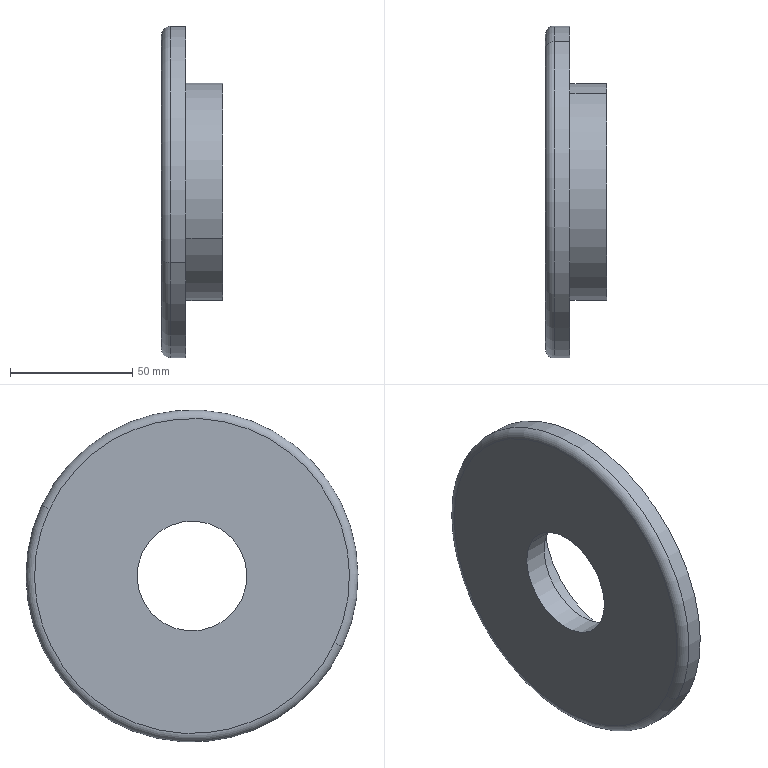Component | SolidWorks | LowerEndCap-1 | 1 solid | 14 faces | box 25 x 136 x 136 mm | volume 155302 mm3 | cylinder 8 | plane 4 | torus 2 | commonest cylinder face diameters 45 x2 75 x2 89 x2 136 x2
build123d program:
from build123d import *


with BuildPart() as part:
    # Sketch1 → Revolve1 (revolve)
    with BuildSketch(Plane(origin=(0, 0, 0), x_dir=(0, 0, -1), z_dir=(1, 0, 0)), mode=Mode.PRIVATE) as revolve1_sk:
        with BuildLine():
            Line((22.5, -10), (64.5, -10))
            ThreePointArc((64.5, -10), (66.975, -8.975), (68, -6.5))
            Line((68, -6.5), (68, 0))
            Line((68, 0), (44.5, 0))
            Line((44.5, 0), (44.5, 15))
            Line((44.5, 15), (37.5, 15))
            Line((37.5, 15), (37.5, 0))
            Line((37.5, 0), (22.5, 0))
            Line((22.5, 0), (22.5, -10))
        make_face()
    revolve(revolve1_sk.sketch.rotate(Axis((0, 0, 0), (0, -1, 0)), 180), axis=Axis((0, 0, 0), (0, -1, 0)))


solid = part.part

# Placed as in the assembly
solid = solid.moved(Location((587.733, 15.31, -110), (0, 0, -90)))
STEP:
#1=COLOUR_RGB('',0.7922,0.8196,0.9333);
#2=FILL_AREA_STYLE_COLOUR('',#1);
#3=FILL_AREA_STYLE('',(#2));
#4=SURFACE_STYLE_FILL_AREA(#3);
#5=SURFACE_SIDE_STYLE('',(#4));
#6=SURFACE_STYLE_USAGE(.BOTH.,#5);
#7=PRESENTATION_STYLE_ASSIGNMENT((#6));
#8=CARTESIAN_POINT('',(22.745,1.405,-3.955));
#9=VERTEX_POINT('',#8);
#10=CARTESIAN_POINT('',(22.745,-0.1993,-4.707));
#11=VERTEX_POINT('',#10);
#12=CARTESIAN_POINT('',(22.745,0.6028,-4.331));
#13=DIRECTION('',(1.,0.,0.));
#14=DIRECTION('',(0.,-0.9054,-0.4246));
#15=AXIS2_PLACEMENT_3D('',#12,#13,#14);
#16=CIRCLE('',#15,0.8858);
#17=EDGE_CURVE('',#9,#11,#16,.T.);
#18=ORIENTED_EDGE('',*,*,#17,.F.);
#19=CARTESIAN_POINT('',(23.139,1.405,-3.955));
#20=VERTEX_POINT('',#19);
#21=CARTESIAN_POINT('',(23.139,1.405,-3.955));
#22=DIRECTION('',(1.,0.,0.));
#23=VECTOR('',#22,39.37);
#24=LINE('',#21,#23);
#25=EDGE_CURVE('',#9,#20,#24,.T.);
#26=ORIENTED_EDGE('',*,*,#25,.T.);
#27=CARTESIAN_POINT('',(23.139,-0.1993,-4.707));
#28=VERTEX_POINT('',#27);
#29=CARTESIAN_POINT('',(23.139,0.6028,-4.331));
#30=DIRECTION('',(1.,0.,0.));
#31=DIRECTION('',(0.,-0.9054,-0.4246));
#32=AXIS2_PLACEMENT_3D('',#29,#30,#31);
#33=CIRCLE('',#32,0.8858);
#34=EDGE_CURVE('',#20,#28,#33,.T.);
#35=ORIENTED_EDGE('',*,*,#34,.T.);
#36=CARTESIAN_POINT('',(23.139,-0.1993,-4.707));
#37=DIRECTION('',(1.,0.,0.));
#38=VECTOR('',#37,39.37);
#39=LINE('',#36,#38);
#40=EDGE_CURVE('',#11,#28,#39,.T.);
#41=ORIENTED_EDGE('',*,*,#40,.F.);
#42=EDGE_LOOP('',(#18,#26,#35,#41));
#43=FACE_OUTER_BOUND('',#42,.T.);
#44=CARTESIAN_POINT('',(23.139,0.6028,-4.331));
#45=DIRECTION('',(1.,0.,0.));
#46=DIRECTION('',(0.,-0.9054,-0.4246));
#47=AXIS2_PLACEMENT_3D('',#44,#45,#46);
#48=CYLINDRICAL_SURFACE('',#47,0.8858);
#49=ADVANCED_FACE('',(#43),#48,.F.);
#50=CARTESIAN_POINT('',(23.139,1.939,-3.704));
#51=VERTEX_POINT('',#50);
#52=CARTESIAN_POINT('',(23.139,-0.7339,-4.958));
#53=VERTEX_POINT('',#52);
#54=CARTESIAN_POINT('',(23.139,0.6028,-4.331));
#55=DIRECTION('',(1.,0.,0.));
#56=DIRECTION('',(0.,-0.9054,-0.4246));
#57=AXIS2_PLACEMENT_3D('',#54,#55,#56);
#58=CIRCLE('',#57,1.476);
#59=EDGE_CURVE('',#51,#53,#58,.T.);
#60=ORIENTED_EDGE('',*,*,#59,.F.);
#61=CARTESIAN_POINT('',(23.73,1.939,-3.704));
#62=VERTEX_POINT('',#61);
#63=CARTESIAN_POINT('',(23.139,1.939,-3.704));
#64=DIRECTION('',(1.,0.,0.));
#65=VECTOR('',#64,39.37);
#66=LINE('',#63,#65);
#67=EDGE_CURVE('',#51,#62,#66,.T.);
#68=ORIENTED_EDGE('',*,*,#67,.T.);
#69=CARTESIAN_POINT('',(23.73,-0.7339,-4.958));
#70=VERTEX_POINT('',#69);
#71=CARTESIAN_POINT('',(23.73,0.6028,-4.331));
#72=DIRECTION('',(1.,0.,0.));
#73=DIRECTION('',(0.,-0.9054,-0.4246));
#74=AXIS2_PLACEMENT_3D('',#71,#72,#73);
#75=CIRCLE('',#74,1.476);
#76=EDGE_CURVE('',#62,#70,#75,.T.);
#77=ORIENTED_EDGE('',*,*,#76,.T.);
#78=CARTESIAN_POINT('',(23.139,-0.7339,-4.958));
#79=DIRECTION('',(1.,0.,0.));
#80=VECTOR('',#79,39.37);
#81=LINE('',#78,#80);
#82=EDGE_CURVE('',#53,#70,#81,.T.);
#83=ORIENTED_EDGE('',*,*,#82,.F.);
#84=EDGE_LOOP('',(#60,#68,#77,#83));
#85=FACE_OUTER_BOUND('',#84,.T.);
#86=CARTESIAN_POINT('',(23.139,0.6028,-4.331));
#87=DIRECTION('',(1.,0.,0.));
#88=DIRECTION('',(0.,-0.9054,-0.4246));
#89=AXIS2_PLACEMENT_3D('',#86,#87,#88);
#90=CYLINDRICAL_SURFACE('',#89,1.476);
#91=ADVANCED_FACE('',(#85),#90,.F.);
#92=CARTESIAN_POINT('',(23.139,-0.9835,-5.075));
#93=VERTEX_POINT('',#92);
#94=CARTESIAN_POINT('',(23.139,2.189,-3.587));
#95=VERTEX_POINT('',#94);
#96=CARTESIAN_POINT('',(23.139,0.6028,-4.331));
#97=DIRECTION('',(1.,0.,0.));
#98=DIRECTION('',(0.,-0.9054,-0.4246));
#99=AXIS2_PLACEMENT_3D('',#96,#97,#98);
#100=CIRCLE('',#99,1.752);
#101=EDGE_CURVE('',#93,#95,#100,.T.);
#102=ORIENTED_EDGE('',*,*,#101,.T.);
#103=CARTESIAN_POINT('',(23.73,2.189,-3.587));
#104=VERTEX_POINT('',#103);
#105=CARTESIAN_POINT('',(23.139,2.189,-3.587));
#106=DIRECTION('',(1.,0.,0.));
#107=VECTOR('',#106,39.37);
#108=LINE('',#105,#107);
#109=EDGE_CURVE('',#95,#104,#108,.T.);
#110=ORIENTED_EDGE('',*,*,#109,.T.);
#111=CARTESIAN_POINT('',(23.73,-0.9835,-5.075));
#112=VERTEX_POINT('',#111);
#113=CARTESIAN_POINT('',(23.73,0.6028,-4.331));
#114=DIRECTION('',(1.,0.,0.));
#115=DIRECTION('',(0.,-0.9054,-0.4246));
#116=AXIS2_PLACEMENT_3D('',#113,#114,#115);
#117=CIRCLE('',#116,1.752);
#118=EDGE_CURVE('',#112,#104,#117,.T.);
#119=ORIENTED_EDGE('',*,*,#118,.F.);
#120=CARTESIAN_POINT('',(23.139,-0.9835,-5.075));
#121=DIRECTION('',(1.,0.,0.));
#122=VECTOR('',#121,39.37);
#123=LINE('',#120,#122);
#124=EDGE_CURVE('',#93,#112,#123,.T.);
#125=ORIENTED_EDGE('',*,*,#124,.F.);
#126=EDGE_LOOP('',(#102,#110,#119,#125));
#127=FACE_OUTER_BOUND('',#126,.T.);
#128=CARTESIAN_POINT('',(23.139,0.6028,-4.331));
#129=DIRECTION('',(1.,0.,0.));
#130=DIRECTION('',(0.,-0.9054,-0.4246));
#131=AXIS2_PLACEMENT_3D('',#128,#129,#130);
#132=CYLINDRICAL_SURFACE('',#131,1.752);
#133=ADVANCED_FACE('',(#127),#132,.T.);
#134=CARTESIAN_POINT('',(22.883,-1.821,-5.467));
#135=VERTEX_POINT('',#134);
#136=CARTESIAN_POINT('',(22.883,3.027,-3.194));
#137=VERTEX_POINT('',#136);
#138=CARTESIAN_POINT('',(22.883,0.6028,-4.331));
#139=DIRECTION('',(1.,0.,0.));
#140=DIRECTION('',(0.,-0.9054,-0.4246));
#141=AXIS2_PLACEMENT_3D('',#138,#139,#140);
#142=CIRCLE('',#141,2.677);
#143=EDGE_CURVE('',#135,#137,#142,.T.);
#144=ORIENTED_EDGE('',*,*,#143,.T.);
#145=CARTESIAN_POINT('',(23.139,3.027,-3.194));
#146=VERTEX_POINT('',#145);
#147=CARTESIAN_POINT('',(23.139,3.027,-3.194));
#148=DIRECTION('',(1.,0.,0.));
#149=VECTOR('',#148,39.37);
#150=LINE('',#147,#149);
#151=EDGE_CURVE('',#137,#146,#150,.T.);
#152=ORIENTED_EDGE('',*,*,#151,.T.);
#153=CARTESIAN_POINT('',(23.139,-1.821,-5.467));
#154=VERTEX_POINT('',#153);
#155=CARTESIAN_POINT('',(23.139,0.6028,-4.331));
#156=DIRECTION('',(1.,0.,0.));
#157=DIRECTION('',(0.,-0.9054,-0.4246));
#158=AXIS2_PLACEMENT_3D('',#155,#156,#157);
#159=CIRCLE('',#158,2.677);
#160=EDGE_CURVE('',#154,#146,#159,.T.);
#161=ORIENTED_EDGE('',*,*,#160,.F.);
#162=CARTESIAN_POINT('',(23.139,-1.821,-5.467));
#163=DIRECTION('',(1.,0.,0.));
#164=VECTOR('',#163,39.37);
#165=LINE('',#162,#164);
#166=EDGE_CURVE('',#135,#154,#165,.T.);
#167=ORIENTED_EDGE('',*,*,#166,.F.);
#168=EDGE_LOOP('',(#144,#152,#161,#167));
#169=FACE_OUTER_BOUND('',#168,.T.);
#170=CARTESIAN_POINT('',(23.139,0.6028,-4.331));
#171=DIRECTION('',(1.,0.,0.));
#172=DIRECTION('',(0.,-0.9054,-0.4246));
#173=AXIS2_PLACEMENT_3D('',#170,#171,#172);
#174=CYLINDRICAL_SURFACE('',#173,2.677);
#175=ADVANCED_FACE('',(#169),#174,.T.);
#176=CARTESIAN_POINT('',(22.745,-1.696,-5.409));
#177=VERTEX_POINT('',#176);
#178=CARTESIAN_POINT('',(22.745,2.902,-3.253));
#179=VERTEX_POINT('',#178);
#180=CARTESIAN_POINT('',(22.745,0.6028,-4.331));
#181=DIRECTION('',(1.,0.,0.));
#182=DIRECTION('',(0.,-0.9054,-0.4246));
#183=AXIS2_PLACEMENT_3D('',#180,#181,#182);
#184=CIRCLE('',#183,2.539);
#185=EDGE_CURVE('',#177,#179,#184,.T.);
#186=ORIENTED_EDGE('',*,*,#185,.T.);
#187=CARTESIAN_POINT('',(22.883,2.902,-3.253));
#188=DIRECTION('',(-0.,0.4246,-0.9054));
#189=DIRECTION('',(0.,0.9054,0.4246));
#190=AXIS2_PLACEMENT_3D('',#187,#188,#189);
#191=CIRCLE('',#190,0.1378);
#192=EDGE_CURVE('',#179,#137,#191,.T.);
#193=ORIENTED_EDGE('',*,*,#192,.T.);
#194=ORIENTED_EDGE('',*,*,#143,.F.);
#195=CARTESIAN_POINT('',(22.883,-1.696,-5.409));
#196=DIRECTION('',(0.,-0.4246,0.9054));
#197=DIRECTION('',(0.,-0.9054,-0.4246));
#198=AXIS2_PLACEMENT_3D('',#195,#196,#197);
#199=CIRCLE('',#198,0.1378);
#200=EDGE_CURVE('',#177,#135,#199,.T.);
#201=ORIENTED_EDGE('',*,*,#200,.F.);
#202=EDGE_LOOP('',(#186,#193,#194,#201));
#203=FACE_OUTER_BOUND('',#202,.T.);
#204=CARTESIAN_POINT('',(22.883,0.6028,-4.331));
#205=DIRECTION('',(1.,0.,0.));
#206=DIRECTION('',(0.,-0.9054,-0.4246));
#207=AXIS2_PLACEMENT_3D('',#204,#205,#206);
#208=TOROIDAL_SURFACE('',#207,2.539,0.1378);
#209=ADVANCED_FACE('',(#203),#208,.T.);
#210=ORIENTED_EDGE('',*,*,#185,.F.);
#211=CARTESIAN_POINT('',(22.745,0.6028,-4.331));
#212=DIRECTION('',(1.,0.,0.));
#213=DIRECTION('',(0.,-0.9054,-0.4246));
#214=AXIS2_PLACEMENT_3D('',#211,#212,#213);
#215=CIRCLE('',#214,2.539);
#216=EDGE_CURVE('',#179,#177,#215,.T.);
#217=ORIENTED_EDGE('',*,*,#216,.F.);
#218=EDGE_LOOP('',(#210,#217));
#219=FACE_OUTER_BOUND('',#218,.T.);
#220=CARTESIAN_POINT('',(22.745,0.6028,-4.331));
#221=DIRECTION('',(1.,0.,0.));
#222=DIRECTION('',(0.,-0.9054,-0.4246));
#223=AXIS2_PLACEMENT_3D('',#220,#221,#222);
#224=CIRCLE('',#223,0.8858);
#225=EDGE_CURVE('',#11,#9,#224,.T.);
#226=ORIENTED_EDGE('',*,*,#225,.T.);
#227=ORIENTED_EDGE('',*,*,#17,.T.);
#228=EDGE_LOOP('',(#226,#227));
#229=FACE_BOUND('',#228,.T.);
#230=CARTESIAN_POINT('',(22.745,0.6028,-4.331));
#231=DIRECTION('',(1.,0.,0.));
#232=DIRECTION('',(0.,-0.9054,-0.4246));
#233=AXIS2_PLACEMENT_3D('',#230,#231,#232);
#234=PLANE('',#233);
#235=ADVANCED_FACE('',(#219,#229),#234,.F.);
#236=ORIENTED_EDGE('',*,*,#192,.F.);
#237=ORIENTED_EDGE('',*,*,#216,.T.);
#238=ORIENTED_EDGE('',*,*,#200,.T.);
#239=CARTESIAN_POINT('',(22.883,0.6028,-4.331));
#240=DIRECTION('',(1.,0.,0.));
#241=DIRECTION('',(0.,-0.9054,-0.4246));
#242=AXIS2_PLACEMENT_3D('',#239,#240,#241);
#243=CIRCLE('',#242,2.677);
#244=EDGE_CURVE('',#137,#135,#243,.T.);
#245=ORIENTED_EDGE('',*,*,#244,.F.);
#246=EDGE_LOOP('',(#236,#237,#238,#245));
#247=FACE_OUTER_BOUND('',#246,.T.);
#248=CARTESIAN_POINT('',(22.883,0.6028,-4.331));
#249=DIRECTION('',(1.,0.,0.));
#250=DIRECTION('',(0.,-0.9054,-0.4246));
#251=AXIS2_PLACEMENT_3D('',#248,#249,#250);
#252=TOROIDAL_SURFACE('',#251,2.539,0.1378);
#253=ADVANCED_FACE('',(#247),#252,.T.);
#254=ORIENTED_EDGE('',*,*,#151,.F.);
#255=ORIENTED_EDGE('',*,*,#244,.T.);
#256=ORIENTED_EDGE('',*,*,#166,.T.);
#257=CARTESIAN_POINT('',(23.139,0.6028,-4.331));
#258=DIRECTION('',(1.,0.,0.));
#259=DIRECTION('',(0.,-0.9054,-0.4246));
#260=AXIS2_PLACEMENT_3D('',#257,#258,#259);
#261=CIRCLE('',#260,2.677);
#262=EDGE_CURVE('',#146,#154,#261,.T.);
#263=ORIENTED_EDGE('',*,*,#262,.F.);
#264=EDGE_LOOP('',(#254,#255,#256,#263));
#265=FACE_OUTER_BOUND('',#264,.T.);
#266=CARTESIAN_POINT('',(23.139,0.6028,-4.331));
#267=DIRECTION('',(1.,0.,0.));
#268=DIRECTION('',(0.,-0.9054,-0.4246));
#269=AXIS2_PLACEMENT_3D('',#266,#267,#268);
#270=CYLINDRICAL_SURFACE('',#269,2.677);
#271=ADVANCED_FACE('',(#265),#270,.T.);
#272=ORIENTED_EDGE('',*,*,#160,.T.);
#273=ORIENTED_EDGE('',*,*,#262,.T.);
#274=EDGE_LOOP('',(#272,#273));
#275=FACE_OUTER_BOUND('',#274,.T.);
#276=ORIENTED_EDGE('',*,*,#101,.F.);
#277=CARTESIAN_POINT('',(23.139,0.6028,-4.331));
#278=DIRECTION('',(1.,0.,0.));
#279=DIRECTION('',(0.,-0.9054,-0.4246));
#280=AXIS2_PLACEMENT_3D('',#277,#278,#279);
#281=CIRCLE('',#280,1.752);
#282=EDGE_CURVE('',#95,#93,#281,.T.);
#283=ORIENTED_EDGE('',*,*,#282,.F.);
#284=EDGE_LOOP('',(#276,#283));
#285=FACE_BOUND('',#284,.T.);
#286=CARTESIAN_POINT('',(23.139,0.6028,-4.331));
#287=DIRECTION('',(1.,0.,0.));
#288=DIRECTION('',(0.,-0.9054,-0.4246));
#289=AXIS2_PLACEMENT_3D('',#286,#287,#288);
#290=PLANE('',#289);
#291=ADVANCED_FACE('',(#275,#285),#290,.T.);
#292=ORIENTED_EDGE('',*,*,#109,.F.);
#293=ORIENTED_EDGE('',*,*,#282,.T.);
#294=ORIENTED_EDGE('',*,*,#124,.T.);
#295=CARTESIAN_POINT('',(23.73,0.6028,-4.331));
#296=DIRECTION('',(1.,0.,0.));
#297=DIRECTION('',(0.,-0.9054,-0.4246));
#298=AXIS2_PLACEMENT_3D('',#295,#296,#297);
#299=CIRCLE('',#298,1.752);
#300=EDGE_CURVE('',#104,#112,#299,.T.);
#301=ORIENTED_EDGE('',*,*,#300,.F.);
#302=EDGE_LOOP('',(#292,#293,#294,#301));
#303=FACE_OUTER_BOUND('',#302,.T.);
#304=CARTESIAN_POINT('',(23.139,0.6028,-4.331));
#305=DIRECTION('',(1.,0.,0.));
#306=DIRECTION('',(0.,-0.9054,-0.4246));
#307=AXIS2_PLACEMENT_3D('',#304,#305,#306);
#308=CYLINDRICAL_SURFACE('',#307,1.752);
#309=ADVANCED_FACE('',(#303),#308,.T.);
#310=ORIENTED_EDGE('',*,*,#118,.T.);
#311=ORIENTED_EDGE('',*,*,#300,.T.);
#312=EDGE_LOOP('',(#310,#311));
#313=FACE_OUTER_BOUND('',#312,.T.);
#314=CARTESIAN_POINT('',(23.73,0.6028,-4.331));
#315=DIRECTION('',(1.,0.,0.));
#316=DIRECTION('',(0.,-0.9054,-0.4246));
#317=AXIS2_PLACEMENT_3D('',#314,#315,#316);
#318=CIRCLE('',#317,1.476);
#319=EDGE_CURVE('',#70,#62,#318,.T.);
#320=ORIENTED_EDGE('',*,*,#319,.F.);
#321=ORIENTED_EDGE('',*,*,#76,.F.);
#322=EDGE_LOOP('',(#320,#321));
#323=FACE_BOUND('',#322,.T.);
#324=CARTESIAN_POINT('',(23.73,0.6028,-4.331));
#325=DIRECTION('',(1.,0.,0.));
#326=DIRECTION('',(0.,-0.9054,-0.4246));
#327=AXIS2_PLACEMENT_3D('',#324,#325,#326);
#328=PLANE('',#327);
#329=ADVANCED_FACE('',(#313,#323),#328,.T.);
#330=ORIENTED_EDGE('',*,*,#67,.F.);
#331=CARTESIAN_POINT('',(23.139,0.6028,-4.331));
#332=DIRECTION('',(1.,0.,0.));
#333=DIRECTION('',(0.,-0.9054,-0.4246));
#334=AXIS2_PLACEMENT_3D('',#331,#332,#333);
#335=CIRCLE('',#334,1.476);
#336=EDGE_CURVE('',#53,#51,#335,.T.);
#337=ORIENTED_EDGE('',*,*,#336,.F.);
#338=ORIENTED_EDGE('',*,*,#82,.T.);
#339=ORIENTED_EDGE('',*,*,#319,.T.);
#340=EDGE_LOOP('',(#330,#337,#338,#339));
#341=FACE_OUTER_BOUND('',#340,.T.);
#342=CARTESIAN_POINT('',(23.139,0.6028,-4.331));
#343=DIRECTION('',(1.,0.,0.));
#344=DIRECTION('',(0.,-0.9054,-0.4246));
#345=AXIS2_PLACEMENT_3D('',#342,#343,#344);
#346=CYLINDRICAL_SURFACE('',#345,1.476);
#347=ADVANCED_FACE('',(#341),#346,.F.);
#348=ORIENTED_EDGE('',*,*,#336,.T.);
#349=ORIENTED_EDGE('',*,*,#59,.T.);
#350=EDGE_LOOP('',(#348,#349));
#351=FACE_OUTER_BOUND('',#350,.T.);
#352=CARTESIAN_POINT('',(23.139,0.6028,-4.331));
#353=DIRECTION('',(1.,0.,0.));
#354=DIRECTION('',(0.,-0.9054,-0.4246));
#355=AXIS2_PLACEMENT_3D('',#352,#353,#354);
#356=CIRCLE('',#355,0.8858);
#357=EDGE_CURVE('',#28,#20,#356,.T.);
#358=ORIENTED_EDGE('',*,*,#357,.F.);
#359=ORIENTED_EDGE('',*,*,#34,.F.);
#360=EDGE_LOOP('',(#358,#359));
#361=FACE_BOUND('',#360,.T.);
#362=CARTESIAN_POINT('',(23.139,0.6028,-4.331));
#363=DIRECTION('',(1.,0.,0.));
#364=DIRECTION('',(0.,-0.9054,-0.4246));
#365=AXIS2_PLACEMENT_3D('',#362,#363,#364);
#366=PLANE('',#365);
#367=ADVANCED_FACE('',(#351,#361),#366,.T.);
#368=ORIENTED_EDGE('',*,*,#25,.F.);
#369=ORIENTED_EDGE('',*,*,#225,.F.);
#370=ORIENTED_EDGE('',*,*,#40,.T.);
#371=ORIENTED_EDGE('',*,*,#357,.T.);
#372=EDGE_LOOP('',(#368,#369,#370,#371));
#373=FACE_OUTER_BOUND('',#372,.T.);
#374=CARTESIAN_POINT('',(23.139,0.6028,-4.331));
#375=DIRECTION('',(1.,0.,0.));
#376=DIRECTION('',(0.,-0.9054,-0.4246));
#377=AXIS2_PLACEMENT_3D('',#374,#375,#376);
#378=CYLINDRICAL_SURFACE('',#377,0.8858);
#379=ADVANCED_FACE('',(#373),#378,.F.);
#380=CLOSED_SHELL('',(#49,#91,#133,#175,#209,#235,#253,#271,#291,#309,#329,#347,#367,#379));
#381=MANIFOLD_SOLID_BREP('',#380);
#382=STYLED_ITEM('',(#7),#381);
#383=PRESENTATION_LAYER_ASSIGNMENT('','',(#382));
#384=(LENGTH_UNIT()NAMED_UNIT(*)SI_UNIT($,.METRE.));
#385=LENGTH_MEASURE_WITH_UNIT(LENGTH_MEASURE(0.0254),#384);
#386=DIMENSIONAL_EXPONENTS(1.,0.,0.,0.,0.,0.,0.);
#387=(CONVERSION_BASED_UNIT('',#385)LENGTH_UNIT()NAMED_UNIT(#386));
#388=UNCERTAINTY_MEASURE_WITH_UNIT(LENGTH_MEASURE(0.00001),#387,'','');
#389=(NAMED_UNIT(*)PLANE_ANGLE_UNIT()SI_UNIT($,.RADIAN.));
#390=(NAMED_UNIT(*)SI_UNIT($,.STERADIAN.)SOLID_ANGLE_UNIT());
#391=(GEOMETRIC_REPRESENTATION_CONTEXT(3)GLOBAL_UNCERTAINTY_ASSIGNED_CONTEXT((#388))GLOBAL_UNIT_ASSIGNED_CONTEXT((#387,#389,#390))REPRESENTATION_CONTEXT('',''));
#392=MECHANICAL_DESIGN_GEOMETRIC_PRESENTATION_REPRESENTATION('',(#382),#391);
#393=CARTESIAN_POINT('',(0.,0.,0.));
#394=DIRECTION('',(0.,0.,1.));
#395=DIRECTION('',(1.,0.,0.));
#396=AXIS2_PLACEMENT_3D('',#393,#394,#395);
#397=(LENGTH_UNIT()NAMED_UNIT(*)SI_UNIT($,.METRE.));
#398=LENGTH_MEASURE_WITH_UNIT(LENGTH_MEASURE(0.0254),#397);
#399=DIMENSIONAL_EXPONENTS(1.,0.,0.,0.,0.,0.,0.);
#400=(CONVERSION_BASED_UNIT('',#398)LENGTH_UNIT()NAMED_UNIT(#399));
#401=UNCERTAINTY_MEASURE_WITH_UNIT(LENGTH_MEASURE(0.00001),#400,'','');
#402=(NAMED_UNIT(*)PLANE_ANGLE_UNIT()SI_UNIT($,.RADIAN.));
#403=(NAMED_UNIT(*)SI_UNIT($,.STERADIAN.)SOLID_ANGLE_UNIT());
#404=(GEOMETRIC_REPRESENTATION_CONTEXT(3)GLOBAL_UNCERTAINTY_ASSIGNED_CONTEXT((#401))GLOBAL_UNIT_ASSIGNED_CONTEXT((#400,#402,#403))REPRESENTATION_CONTEXT('',''));
#405=ADVANCED_BREP_SHAPE_REPRESENTATION('',(#381,#396),#404);